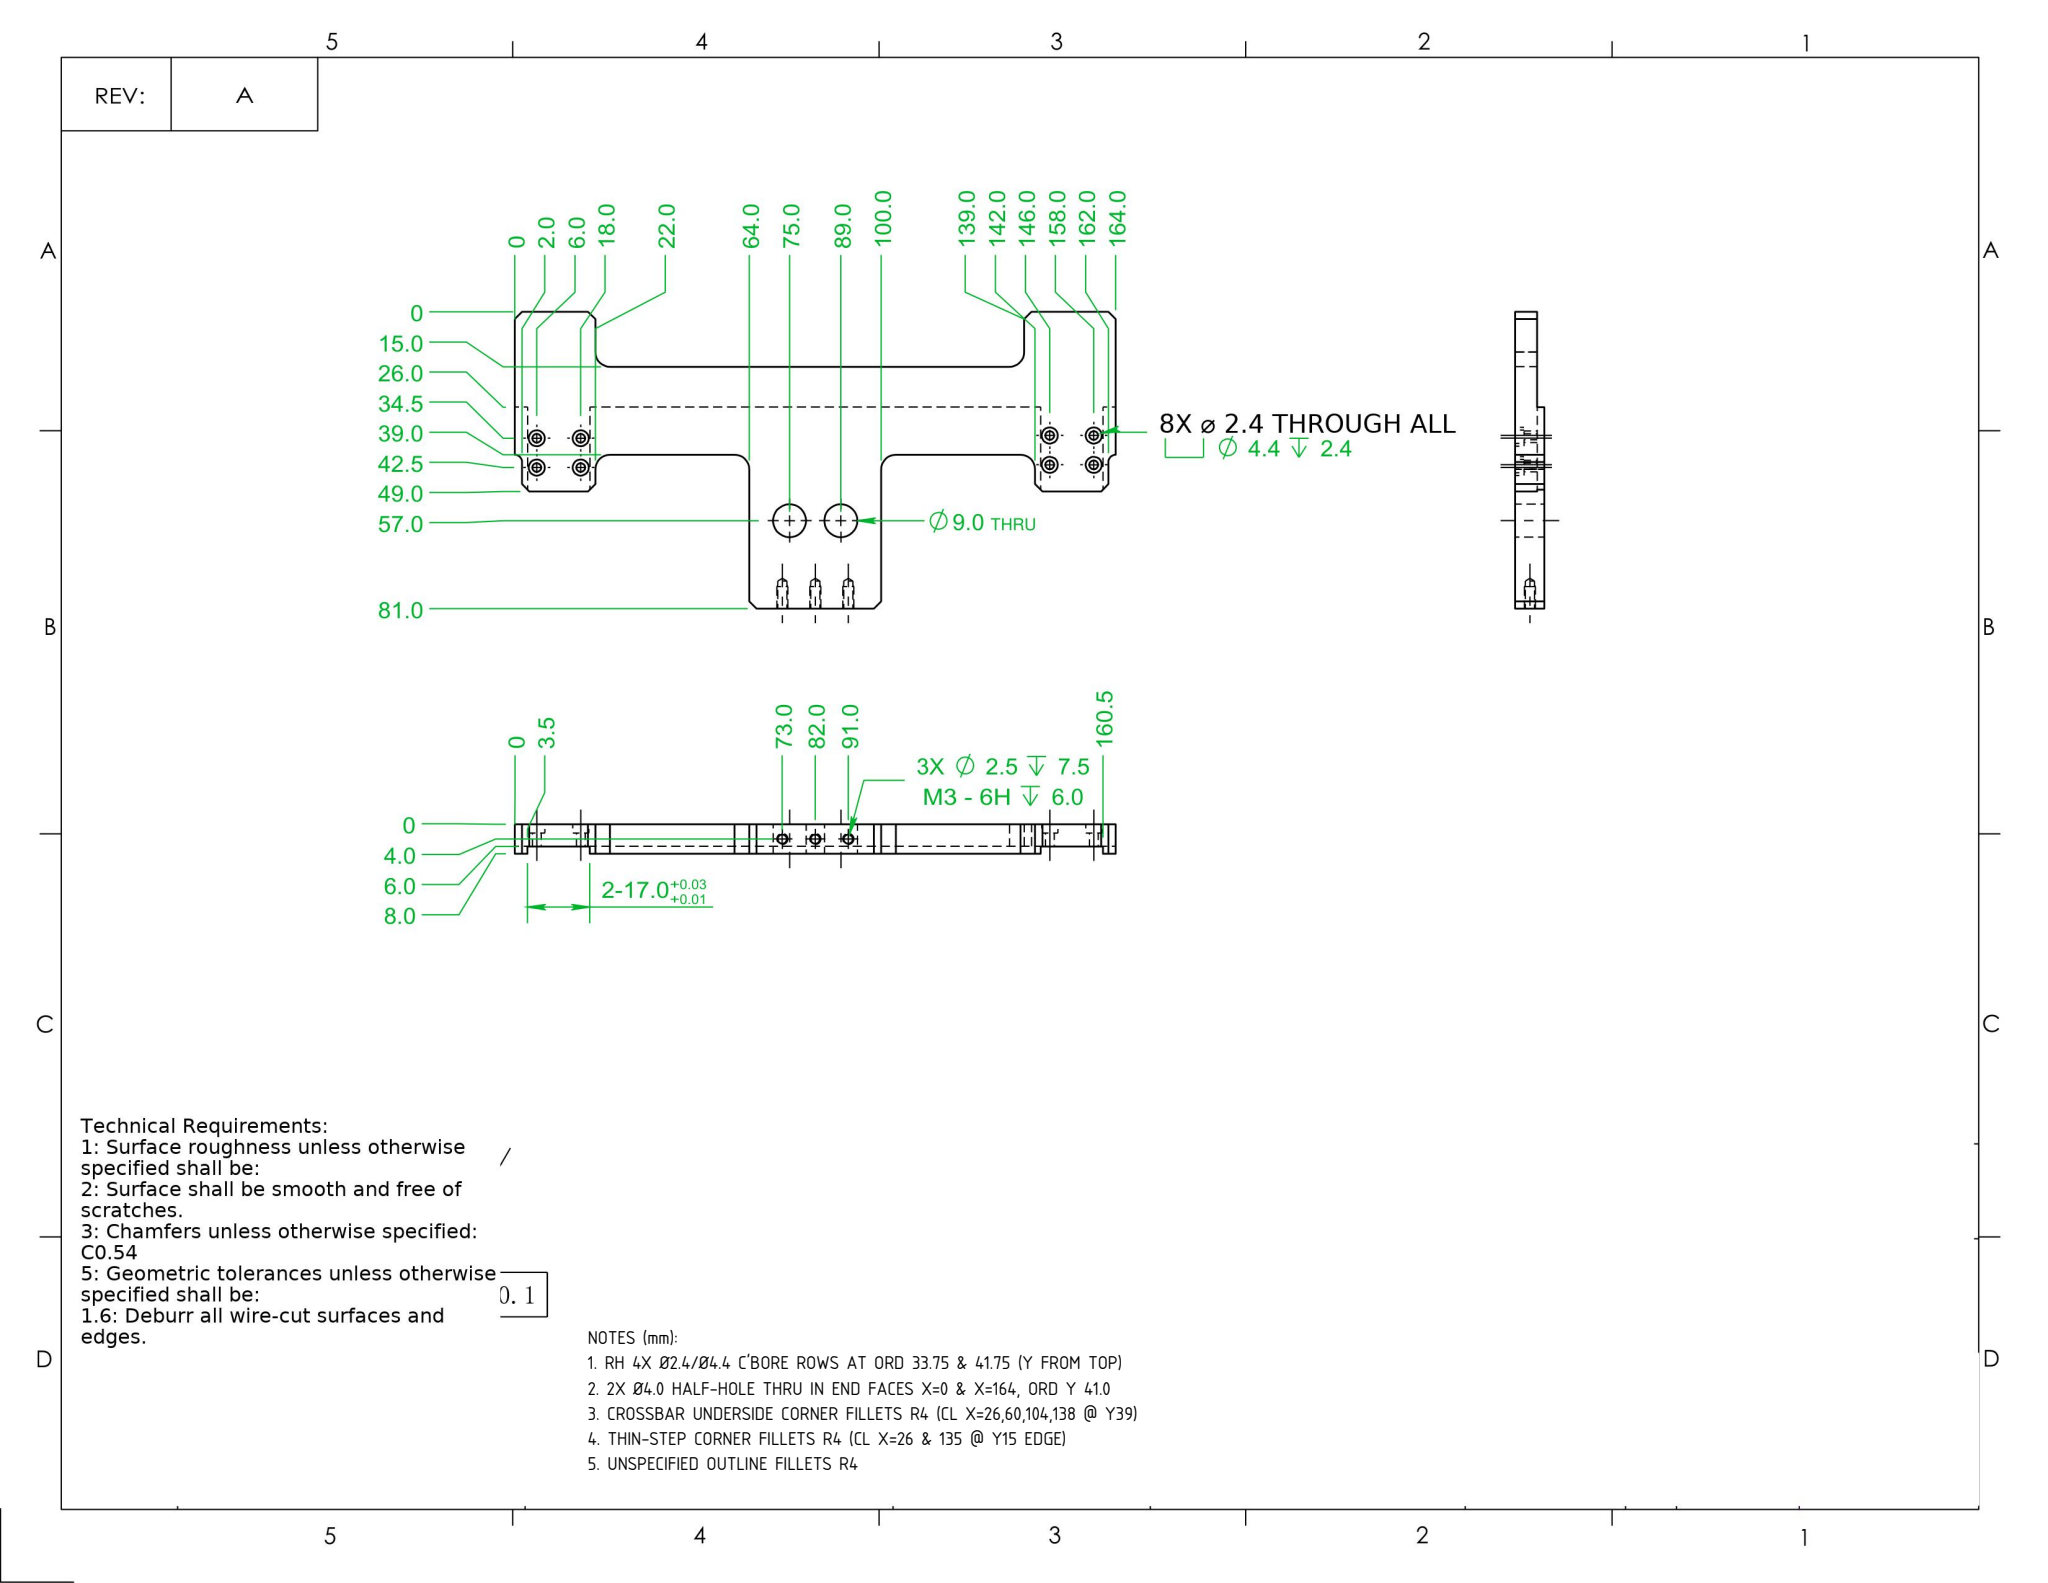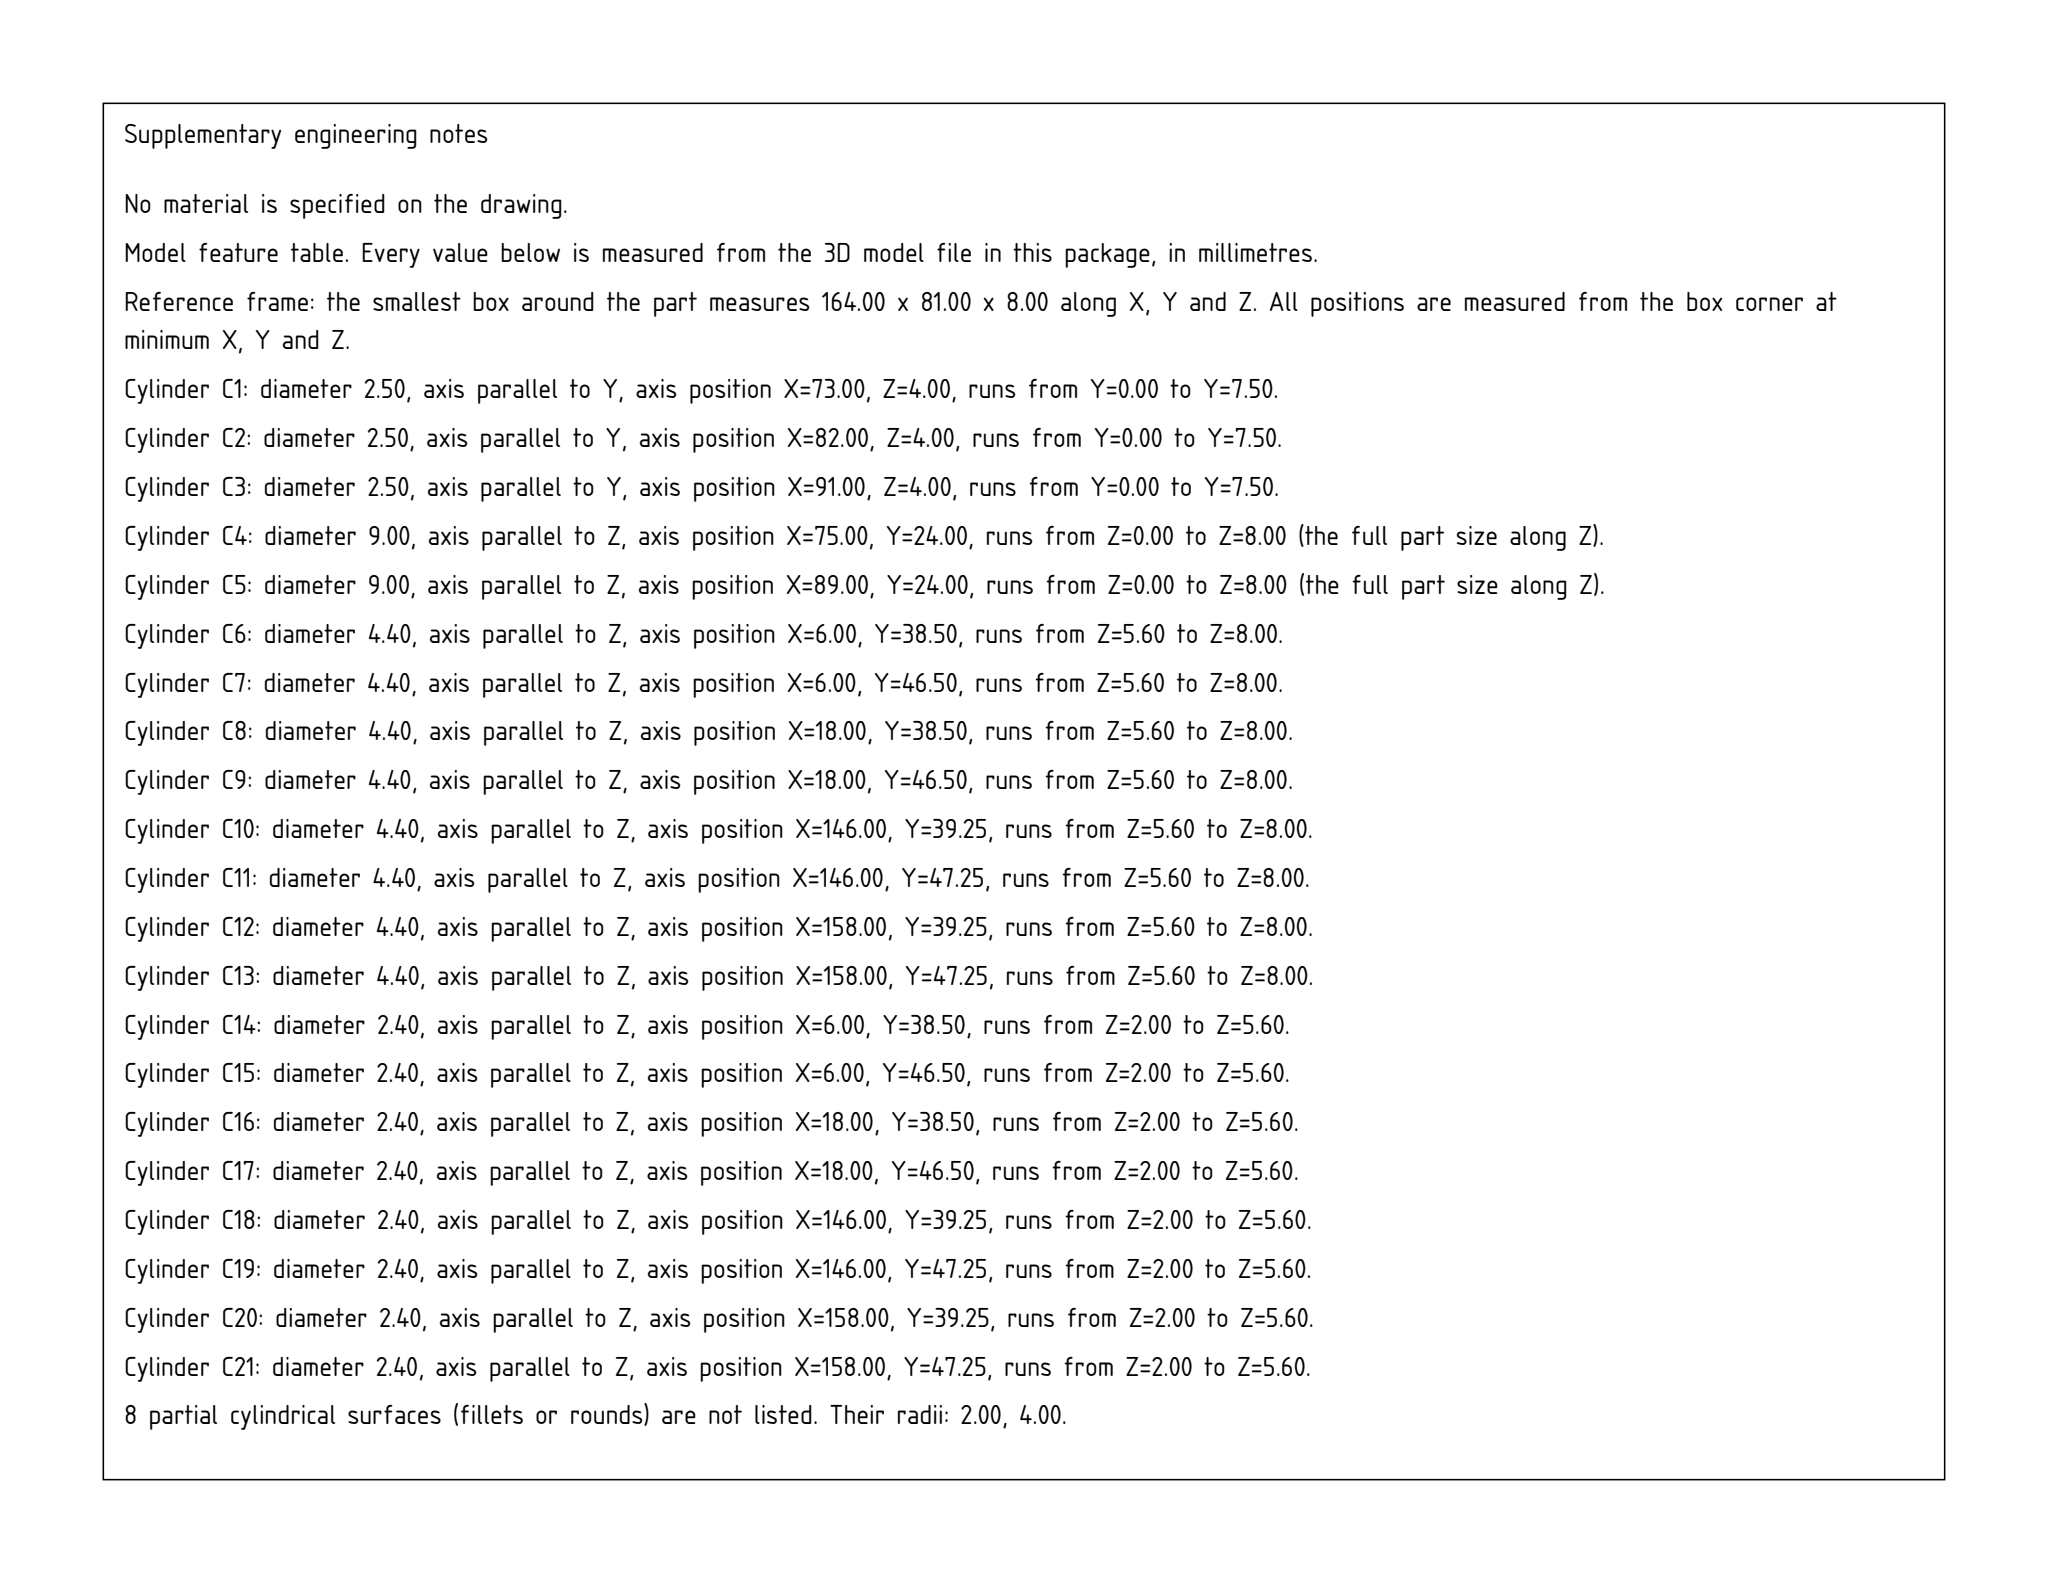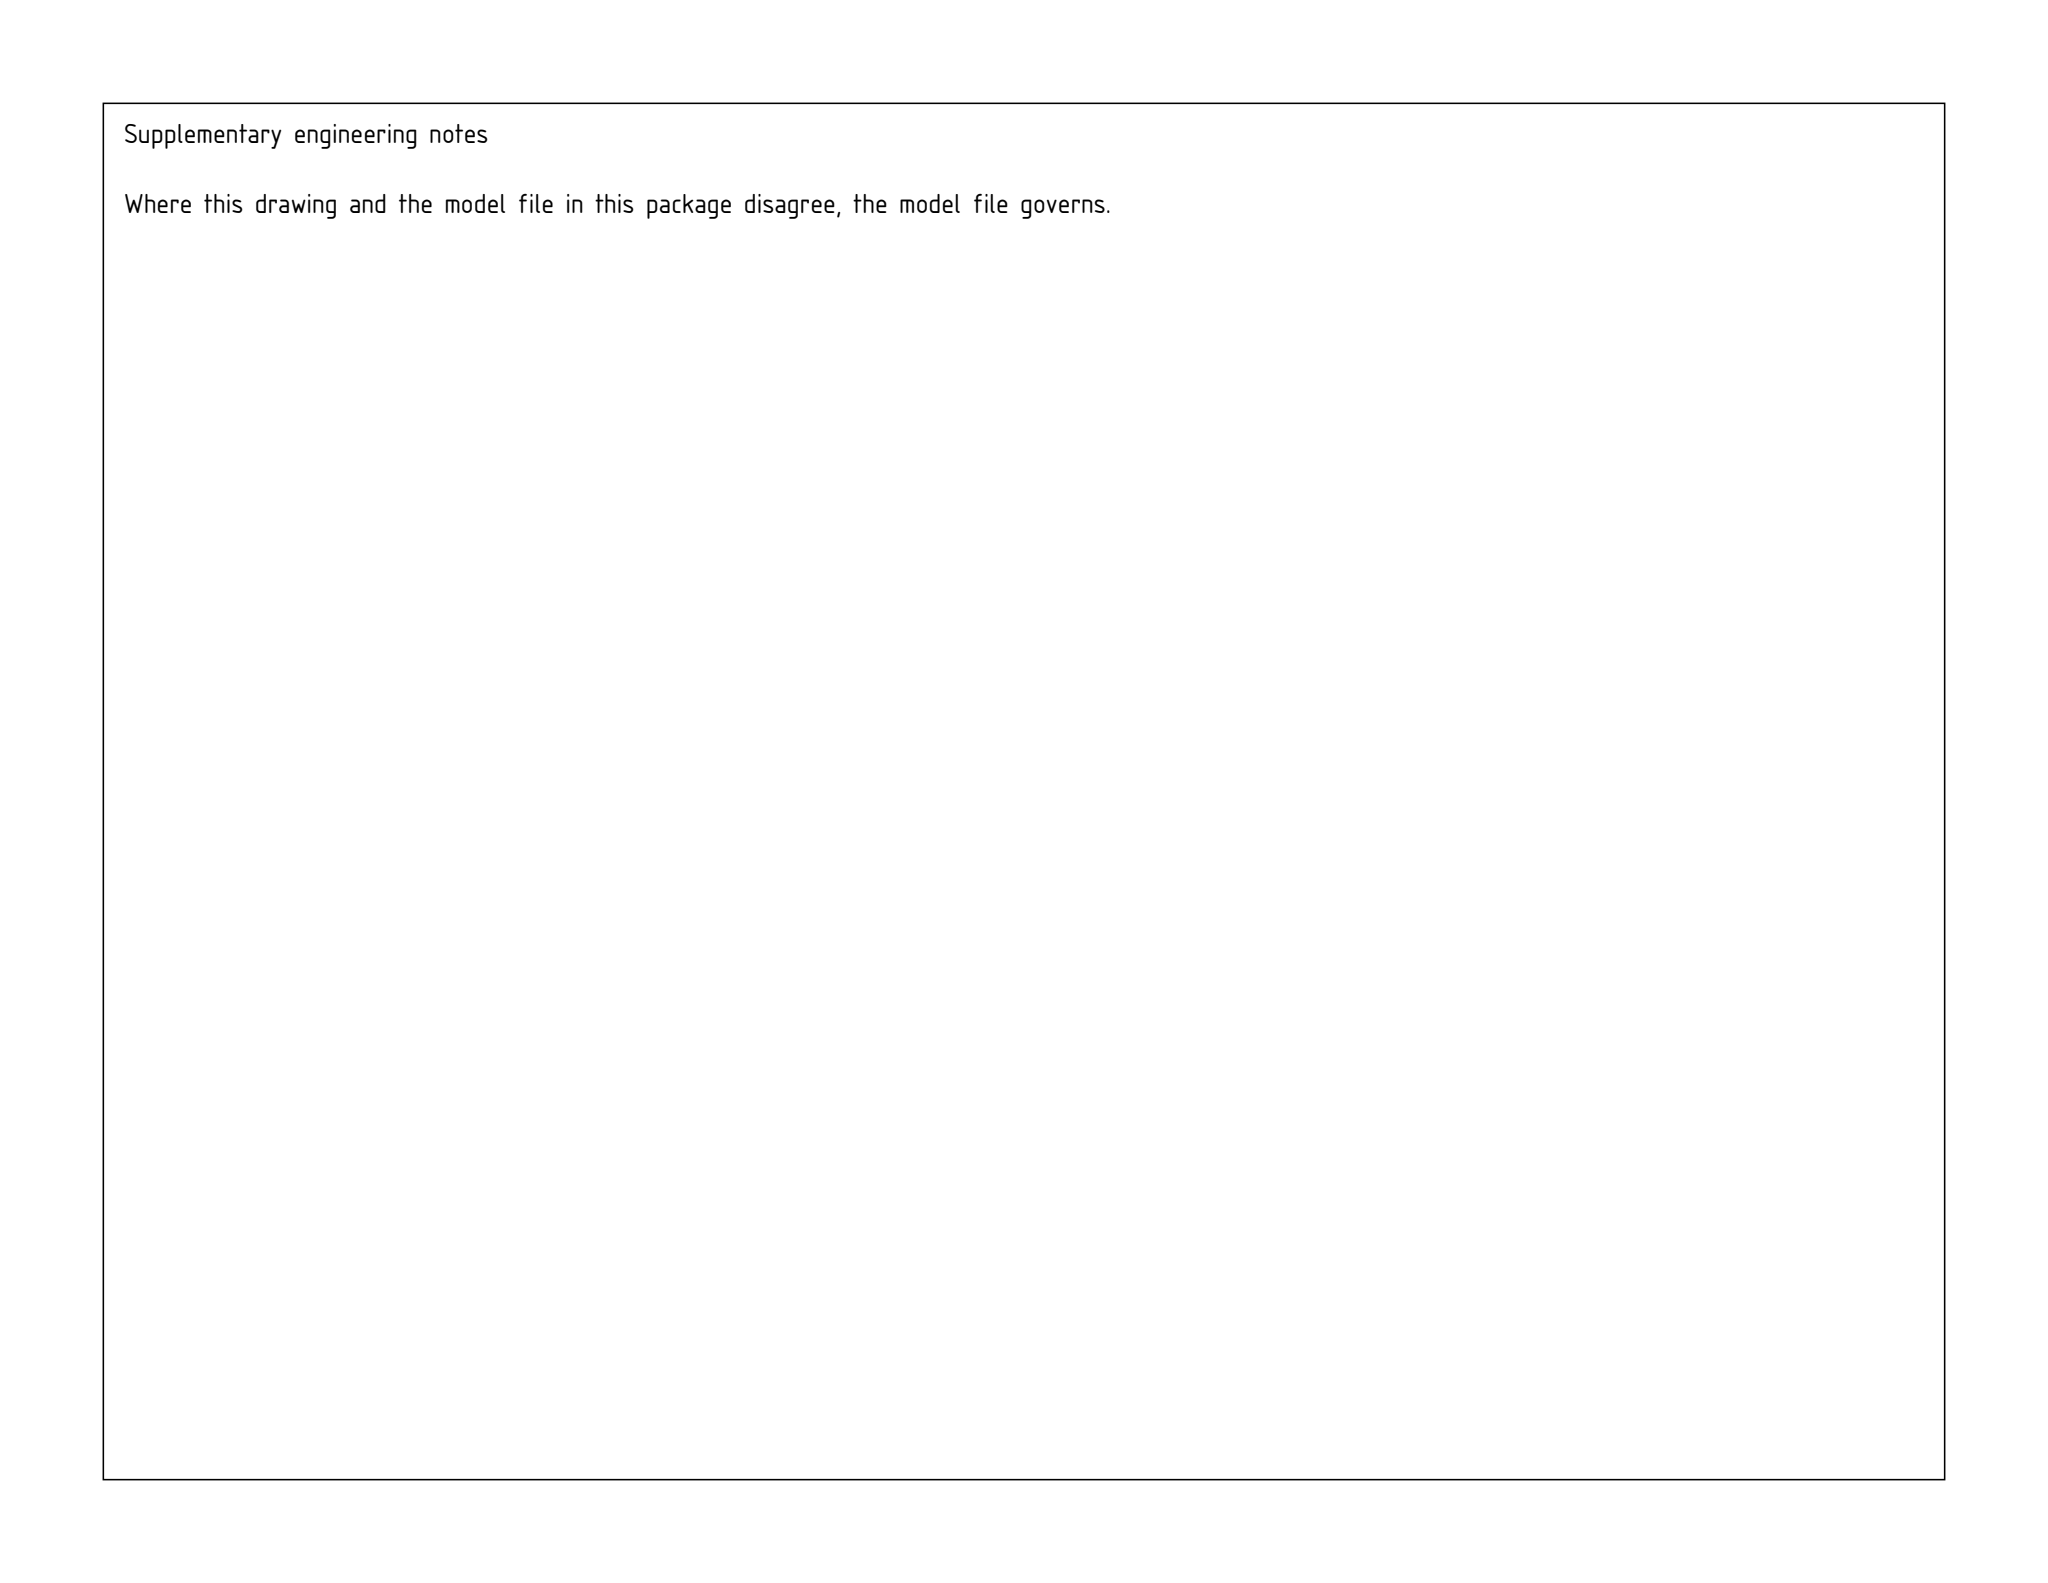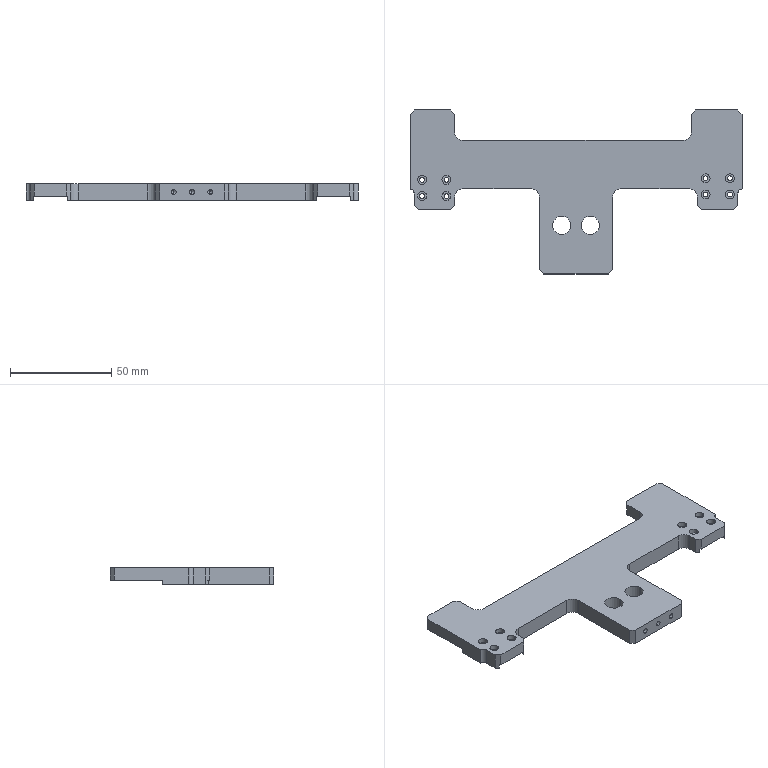Part | SolidWorks | mm | 1 solid | 104 faces | box 164 x 81 x 8 mm | volume 44310 mm3 | cylinder 50 | plane 48 | cone 6 | commonest cylinder face diameters 4.4 x16 2.4 x16 2.5 x6 8 x6 9 x4 4 x2
Drawing notes:
RH 4X Ø2.4/Ø4.4 C'BORE ROWS AT ORD 33.75 & 41.75 (Y FROM TOP) | from the solid: Ø2.4/Ø4.4 z-holes at y=39.25 & 47.25 from bottom; 81-47.25=33.75, 81-39.25=41.75
2X Ø4.0 HALF-HOLE THRU IN END FACES X=0 & X=164, ORD Y 41.0 | from the solid: Ø4.0 z-cylinders, len 8.0 (full thk), at (0,40) and (164,40); 81-40=41.0
CROSSBAR UNDERSIDE CORNER FILLETS R4 (CL X=26,60,104,138 @ Y39) | from the solid: Ø8.0 z-cylinders at (26,38),(60,38),(104,38),(138,38), len 8.0 = full thk -> R4 tangent arcs
THIN-STEP CORNER FILLETS R4 (CL X=26 & 135 @ Y15 EDGE) | from the solid: Ø8.0 z-cylinders at (26,70),(135,70), len 6.0 = step depth -> R4 tangent arcs
UNSPECIFIED OUTLINE FILLETS R4 | from the solid: All outline tangent arcs in STEP are Ø8.0 cylinders -> R4